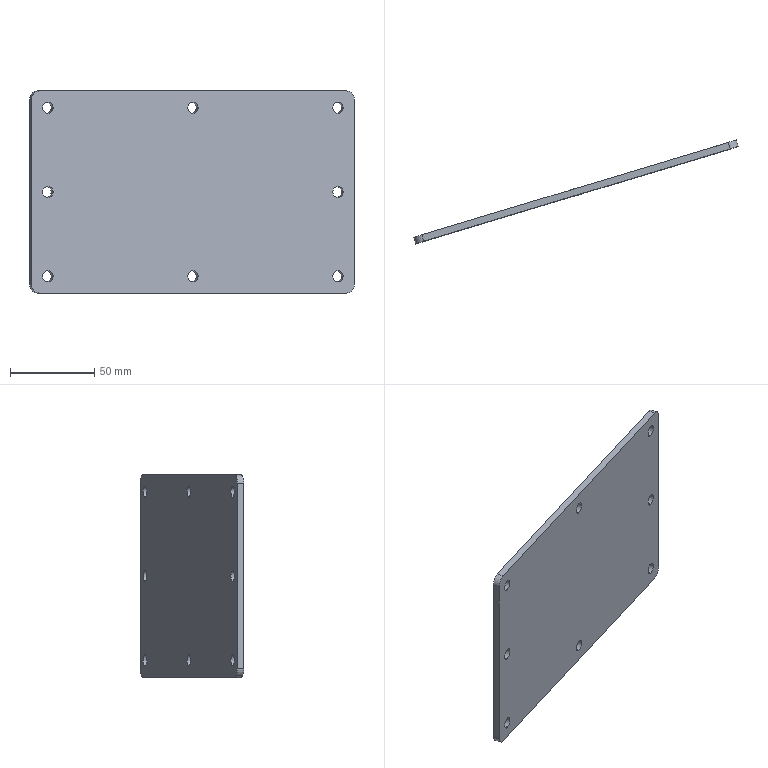Component | SolidWorks | SightHoleCoverA-1 | 1 solid | 26 faces | box 192.63 x 61.61 x 120 mm | volume 94852 mm3 | cylinder 20 | plane 6 | commonest cylinder face diameters 6.5 x16 10 x4
build123d program:
from build123d import *

# Parameters (mm, degrees)
SKETCH1_W                  = 200
SKETCH1_H                  = 120
BOSS_EXTRUDE1_DEPTH        = 4
F_6_5_6_5_DIAMETER_HOLE1_D = 6.5
FILLET1_R                  = 5


with BuildPart() as part:
    # Sketch1 → Boss-Extrude1 (new body)
    with BuildSketch(Plane(origin=(0, 0, 0), x_dir=(1, 0, 0), z_dir=(0, 1, 0))):
        Rectangle(SKETCH1_W, SKETCH1_H)
    extrude(amount=-BOSS_EXTRUDE1_DEPTH)

    # 6.5 _6.5_ Diameter Hole1 (through all)
    with Locations(Plane(origin=(0, -4, 0), x_dir=(-1, 0, 0), z_dir=(0, -1, 0))):
        with Locations((-90, 50), (0, 50), (90, 50), (90, 0), (-90, 0), (-90, -50), (0, -50), (90, -50)):
            Hole(F_6_5_6_5_DIAMETER_HOLE1_D / 2)

    # Fillet1
    fillet1_edges = [part.edges().sort_by_distance(p)[0] for p in [
        (-100, -2, 60),
        (-100, -2, -60),
        (100, -2, -60),
        (100, -2, 60),
    ]]
    fillet(fillet1_edges, radius=FILLET1_R)


solid = part.part

# Placed as in the assembly
solid = solid.moved(Location((-162.617, 165.059, 0), (180, 0, -16.791)))
STEP:
#1=COLOUR_RGB('',0.7922,0.8196,0.9333);
#2=FILL_AREA_STYLE_COLOUR('',#1);
#3=FILL_AREA_STYLE('',(#2));
#4=SURFACE_STYLE_FILL_AREA(#3);
#5=SURFACE_SIDE_STYLE('',(#4));
#6=SURFACE_STYLE_USAGE(.BOTH.,#5);
#7=PRESENTATION_STYLE_ASSIGNMENT((#6));
#8=CARTESIAN_POINT('',(-3.056,7.673,-1.841));
#9=VERTEX_POINT('',#8);
#10=CARTESIAN_POINT('',(-3.056,7.673,-2.096));
#11=VERTEX_POINT('',#10);
#12=CARTESIAN_POINT('',(-3.056,7.673,-1.969));
#13=DIRECTION('',(0.2889,-0.9574,0.));
#14=DIRECTION('',(0.,0.,-1.));
#15=AXIS2_PLACEMENT_3D('',#12,#13,#14);
#16=CIRCLE('',#15,0.128);
#17=EDGE_CURVE('',#9,#11,#16,.T.);
#18=ORIENTED_EDGE('',*,*,#17,.F.);
#19=CARTESIAN_POINT('',(-3.01,7.522,-1.841));
#20=VERTEX_POINT('',#19);
#21=CARTESIAN_POINT('',(-3.01,7.522,-1.841));
#22=DIRECTION('',(0.2889,-0.9574,0.));
#23=VECTOR('',#22,39.37);
#24=LINE('',#21,#23);
#25=EDGE_CURVE('',#9,#20,#24,.T.);
#26=ORIENTED_EDGE('',*,*,#25,.T.);
#27=CARTESIAN_POINT('',(-3.01,7.522,-2.096));
#28=VERTEX_POINT('',#27);
#29=CARTESIAN_POINT('',(-3.01,7.522,-1.969));
#30=DIRECTION('',(0.2889,-0.9574,0.));
#31=DIRECTION('',(0.,0.,-1.));
#32=AXIS2_PLACEMENT_3D('',#29,#30,#31);
#33=CIRCLE('',#32,0.128);
#34=EDGE_CURVE('',#20,#28,#33,.T.);
#35=ORIENTED_EDGE('',*,*,#34,.T.);
#36=CARTESIAN_POINT('',(-3.01,7.522,-2.096));
#37=DIRECTION('',(0.2889,-0.9574,0.));
#38=VECTOR('',#37,39.37);
#39=LINE('',#36,#38);
#40=EDGE_CURVE('',#11,#28,#39,.T.);
#41=ORIENTED_EDGE('',*,*,#40,.F.);
#42=EDGE_LOOP('',(#18,#26,#35,#41));
#43=FACE_OUTER_BOUND('',#42,.T.);
#44=CARTESIAN_POINT('',(-3.01,7.522,-1.969));
#45=DIRECTION('',(0.2889,-0.9574,0.));
#46=DIRECTION('',(0.,0.,-1.));
#47=AXIS2_PLACEMENT_3D('',#44,#45,#46);
#48=CYLINDRICAL_SURFACE('',#47,0.128);
#49=ADVANCED_FACE('',(#43),#48,.F.);
#50=CARTESIAN_POINT('',(-6.448,6.649,-1.841));
#51=VERTEX_POINT('',#50);
#52=CARTESIAN_POINT('',(-6.448,6.649,-2.096));
#53=VERTEX_POINT('',#52);
#54=CARTESIAN_POINT('',(-6.448,6.649,-1.969));
#55=DIRECTION('',(0.2889,-0.9574,0.));
#56=DIRECTION('',(0.,0.,-1.));
#57=AXIS2_PLACEMENT_3D('',#54,#55,#56);
#58=CIRCLE('',#57,0.128);
#59=EDGE_CURVE('',#51,#53,#58,.T.);
#60=ORIENTED_EDGE('',*,*,#59,.F.);
#61=CARTESIAN_POINT('',(-6.402,6.498,-1.841));
#62=VERTEX_POINT('',#61);
#63=CARTESIAN_POINT('',(-6.402,6.498,-1.841));
#64=DIRECTION('',(0.2889,-0.9574,0.));
#65=VECTOR('',#64,39.37);
#66=LINE('',#63,#65);
#67=EDGE_CURVE('',#51,#62,#66,.T.);
#68=ORIENTED_EDGE('',*,*,#67,.T.);
#69=CARTESIAN_POINT('',(-6.402,6.498,-2.096));
#70=VERTEX_POINT('',#69);
#71=CARTESIAN_POINT('',(-6.402,6.498,-1.969));
#72=DIRECTION('',(0.2889,-0.9574,0.));
#73=DIRECTION('',(0.,0.,-1.));
#74=AXIS2_PLACEMENT_3D('',#71,#72,#73);
#75=CIRCLE('',#74,0.128);
#76=EDGE_CURVE('',#62,#70,#75,.T.);
#77=ORIENTED_EDGE('',*,*,#76,.T.);
#78=CARTESIAN_POINT('',(-6.402,6.498,-2.096));
#79=DIRECTION('',(0.2889,-0.9574,0.));
#80=VECTOR('',#79,39.37);
#81=LINE('',#78,#80);
#82=EDGE_CURVE('',#53,#70,#81,.T.);
#83=ORIENTED_EDGE('',*,*,#82,.F.);
#84=EDGE_LOOP('',(#60,#68,#77,#83));
#85=FACE_OUTER_BOUND('',#84,.T.);
#86=CARTESIAN_POINT('',(-6.402,6.498,-1.969));
#87=DIRECTION('',(0.2889,-0.9574,0.));
#88=DIRECTION('',(0.,0.,-1.));
#89=AXIS2_PLACEMENT_3D('',#86,#87,#88);
#90=CYLINDRICAL_SURFACE('',#89,0.128);
#91=ADVANCED_FACE('',(#85),#90,.F.);
#92=CARTESIAN_POINT('',(-9.84,5.626,-1.841));
#93=VERTEX_POINT('',#92);
#94=CARTESIAN_POINT('',(-9.84,5.626,-2.096));
#95=VERTEX_POINT('',#94);
#96=CARTESIAN_POINT('',(-9.84,5.626,-1.969));
#97=DIRECTION('',(0.2889,-0.9574,0.));
#98=DIRECTION('',(0.,0.,-1.));
#99=AXIS2_PLACEMENT_3D('',#96,#97,#98);
#100=CIRCLE('',#99,0.128);
#101=EDGE_CURVE('',#93,#95,#100,.T.);
#102=ORIENTED_EDGE('',*,*,#101,.F.);
#103=CARTESIAN_POINT('',(-9.794,5.475,-1.841));
#104=VERTEX_POINT('',#103);
#105=CARTESIAN_POINT('',(-9.794,5.475,-1.841));
#106=DIRECTION('',(0.2889,-0.9574,0.));
#107=VECTOR('',#106,39.37);
#108=LINE('',#105,#107);
#109=EDGE_CURVE('',#93,#104,#108,.T.);
#110=ORIENTED_EDGE('',*,*,#109,.T.);
#111=CARTESIAN_POINT('',(-9.794,5.475,-2.096));
#112=VERTEX_POINT('',#111);
#113=CARTESIAN_POINT('',(-9.794,5.475,-1.969));
#114=DIRECTION('',(0.2889,-0.9574,0.));
#115=DIRECTION('',(0.,0.,-1.));
#116=AXIS2_PLACEMENT_3D('',#113,#114,#115);
#117=CIRCLE('',#116,0.128);
#118=EDGE_CURVE('',#104,#112,#117,.T.);
#119=ORIENTED_EDGE('',*,*,#118,.T.);
#120=CARTESIAN_POINT('',(-9.794,5.475,-2.096));
#121=DIRECTION('',(0.2889,-0.9574,0.));
#122=VECTOR('',#121,39.37);
#123=LINE('',#120,#122);
#124=EDGE_CURVE('',#95,#112,#123,.T.);
#125=ORIENTED_EDGE('',*,*,#124,.F.);
#126=EDGE_LOOP('',(#102,#110,#119,#125));
#127=FACE_OUTER_BOUND('',#126,.T.);
#128=CARTESIAN_POINT('',(-9.794,5.475,-1.969));
#129=DIRECTION('',(0.2889,-0.9574,0.));
#130=DIRECTION('',(0.,0.,-1.));
#131=AXIS2_PLACEMENT_3D('',#128,#129,#130);
#132=CYLINDRICAL_SURFACE('',#131,0.128);
#133=ADVANCED_FACE('',(#127),#132,.F.);
#134=CARTESIAN_POINT('',(-9.84,5.626,0.128));
#135=VERTEX_POINT('',#134);
#136=CARTESIAN_POINT('',(-9.84,5.626,-0.128));
#137=VERTEX_POINT('',#136);
#138=CARTESIAN_POINT('',(-9.84,5.626,0.));
#139=DIRECTION('',(0.2889,-0.9574,0.));
#140=DIRECTION('',(0.,0.,-1.));
#141=AXIS2_PLACEMENT_3D('',#138,#139,#140);
#142=CIRCLE('',#141,0.128);
#143=EDGE_CURVE('',#135,#137,#142,.T.);
#144=ORIENTED_EDGE('',*,*,#143,.F.);
#145=CARTESIAN_POINT('',(-9.794,5.475,0.128));
#146=VERTEX_POINT('',#145);
#147=CARTESIAN_POINT('',(-9.794,5.475,0.128));
#148=DIRECTION('',(0.2889,-0.9574,0.));
#149=VECTOR('',#148,39.37);
#150=LINE('',#147,#149);
#151=EDGE_CURVE('',#135,#146,#150,.T.);
#152=ORIENTED_EDGE('',*,*,#151,.T.);
#153=CARTESIAN_POINT('',(-9.794,5.475,-0.128));
#154=VERTEX_POINT('',#153);
#155=CARTESIAN_POINT('',(-9.794,5.475,0.));
#156=DIRECTION('',(0.2889,-0.9574,0.));
#157=DIRECTION('',(0.,0.,-1.));
#158=AXIS2_PLACEMENT_3D('',#155,#156,#157);
#159=CIRCLE('',#158,0.128);
#160=EDGE_CURVE('',#146,#154,#159,.T.);
#161=ORIENTED_EDGE('',*,*,#160,.T.);
#162=CARTESIAN_POINT('',(-9.794,5.475,-0.128));
#163=DIRECTION('',(0.2889,-0.9574,0.));
#164=VECTOR('',#163,39.37);
#165=LINE('',#162,#164);
#166=EDGE_CURVE('',#137,#154,#165,.T.);
#167=ORIENTED_EDGE('',*,*,#166,.F.);
#168=EDGE_LOOP('',(#144,#152,#161,#167));
#169=FACE_OUTER_BOUND('',#168,.T.);
#170=CARTESIAN_POINT('',(-9.794,5.475,0.));
#171=DIRECTION('',(0.2889,-0.9574,0.));
#172=DIRECTION('',(0.,0.,-1.));
#173=AXIS2_PLACEMENT_3D('',#170,#171,#172);
#174=CYLINDRICAL_SURFACE('',#173,0.128);
#175=ADVANCED_FACE('',(#169),#174,.F.);
#176=CARTESIAN_POINT('',(-3.056,7.673,0.128));
#177=VERTEX_POINT('',#176);
#178=CARTESIAN_POINT('',(-3.056,7.673,-0.128));
#179=VERTEX_POINT('',#178);
#180=CARTESIAN_POINT('',(-3.056,7.673,0.));
#181=DIRECTION('',(0.2889,-0.9574,0.));
#182=DIRECTION('',(0.,0.,-1.));
#183=AXIS2_PLACEMENT_3D('',#180,#181,#182);
#184=CIRCLE('',#183,0.128);
#185=EDGE_CURVE('',#177,#179,#184,.T.);
#186=ORIENTED_EDGE('',*,*,#185,.F.);
#187=CARTESIAN_POINT('',(-3.01,7.522,0.128));
#188=VERTEX_POINT('',#187);
#189=CARTESIAN_POINT('',(-3.01,7.522,0.128));
#190=DIRECTION('',(0.2889,-0.9574,0.));
#191=VECTOR('',#190,39.37);
#192=LINE('',#189,#191);
#193=EDGE_CURVE('',#177,#188,#192,.T.);
#194=ORIENTED_EDGE('',*,*,#193,.T.);
#195=CARTESIAN_POINT('',(-3.01,7.522,-0.128));
#196=VERTEX_POINT('',#195);
#197=CARTESIAN_POINT('',(-3.01,7.522,0.));
#198=DIRECTION('',(0.2889,-0.9574,0.));
#199=DIRECTION('',(0.,0.,-1.));
#200=AXIS2_PLACEMENT_3D('',#197,#198,#199);
#201=CIRCLE('',#200,0.128);
#202=EDGE_CURVE('',#188,#196,#201,.T.);
#203=ORIENTED_EDGE('',*,*,#202,.T.);
#204=CARTESIAN_POINT('',(-3.01,7.522,-0.128));
#205=DIRECTION('',(0.2889,-0.9574,0.));
#206=VECTOR('',#205,39.37);
#207=LINE('',#204,#206);
#208=EDGE_CURVE('',#179,#196,#207,.T.);
#209=ORIENTED_EDGE('',*,*,#208,.F.);
#210=EDGE_LOOP('',(#186,#194,#203,#209));
#211=FACE_OUTER_BOUND('',#210,.T.);
#212=CARTESIAN_POINT('',(-3.01,7.522,0.));
#213=DIRECTION('',(0.2889,-0.9574,0.));
#214=DIRECTION('',(0.,0.,-1.));
#215=AXIS2_PLACEMENT_3D('',#212,#213,#214);
#216=CYLINDRICAL_SURFACE('',#215,0.128);
#217=ADVANCED_FACE('',(#211),#216,.F.);
#218=CARTESIAN_POINT('',(-3.056,7.673,2.096));
#219=VERTEX_POINT('',#218);
#220=CARTESIAN_POINT('',(-3.056,7.673,1.841));
#221=VERTEX_POINT('',#220);
#222=CARTESIAN_POINT('',(-3.056,7.673,1.969));
#223=DIRECTION('',(0.2889,-0.9574,0.));
#224=DIRECTION('',(0.,0.,-1.));
#225=AXIS2_PLACEMENT_3D('',#222,#223,#224);
#226=CIRCLE('',#225,0.128);
#227=EDGE_CURVE('',#219,#221,#226,.T.);
#228=ORIENTED_EDGE('',*,*,#227,.F.);
#229=CARTESIAN_POINT('',(-3.01,7.522,2.096));
#230=VERTEX_POINT('',#229);
#231=CARTESIAN_POINT('',(-3.01,7.522,2.096));
#232=DIRECTION('',(0.2889,-0.9574,0.));
#233=VECTOR('',#232,39.37);
#234=LINE('',#231,#233);
#235=EDGE_CURVE('',#219,#230,#234,.T.);
#236=ORIENTED_EDGE('',*,*,#235,.T.);
#237=CARTESIAN_POINT('',(-3.01,7.522,1.841));
#238=VERTEX_POINT('',#237);
#239=CARTESIAN_POINT('',(-3.01,7.522,1.969));
#240=DIRECTION('',(0.2889,-0.9574,0.));
#241=DIRECTION('',(0.,0.,-1.));
#242=AXIS2_PLACEMENT_3D('',#239,#240,#241);
#243=CIRCLE('',#242,0.128);
#244=EDGE_CURVE('',#230,#238,#243,.T.);
#245=ORIENTED_EDGE('',*,*,#244,.T.);
#246=CARTESIAN_POINT('',(-3.01,7.522,1.841));
#247=DIRECTION('',(0.2889,-0.9574,0.));
#248=VECTOR('',#247,39.37);
#249=LINE('',#246,#248);
#250=EDGE_CURVE('',#221,#238,#249,.T.);
#251=ORIENTED_EDGE('',*,*,#250,.F.);
#252=EDGE_LOOP('',(#228,#236,#245,#251));
#253=FACE_OUTER_BOUND('',#252,.T.);
#254=CARTESIAN_POINT('',(-3.01,7.522,1.969));
#255=DIRECTION('',(0.2889,-0.9574,0.));
#256=DIRECTION('',(0.,0.,-1.));
#257=AXIS2_PLACEMENT_3D('',#254,#255,#256);
#258=CYLINDRICAL_SURFACE('',#257,0.128);
#259=ADVANCED_FACE('',(#253),#258,.F.);
#260=CARTESIAN_POINT('',(-6.448,6.649,2.096));
#261=VERTEX_POINT('',#260);
#262=CARTESIAN_POINT('',(-6.448,6.649,1.841));
#263=VERTEX_POINT('',#262);
#264=CARTESIAN_POINT('',(-6.448,6.649,1.969));
#265=DIRECTION('',(0.2889,-0.9574,0.));
#266=DIRECTION('',(0.,0.,-1.));
#267=AXIS2_PLACEMENT_3D('',#264,#265,#266);
#268=CIRCLE('',#267,0.128);
#269=EDGE_CURVE('',#261,#263,#268,.T.);
#270=ORIENTED_EDGE('',*,*,#269,.F.);
#271=CARTESIAN_POINT('',(-6.402,6.498,2.096));
#272=VERTEX_POINT('',#271);
#273=CARTESIAN_POINT('',(-6.402,6.498,2.096));
#274=DIRECTION('',(0.2889,-0.9574,0.));
#275=VECTOR('',#274,39.37);
#276=LINE('',#273,#275);
#277=EDGE_CURVE('',#261,#272,#276,.T.);
#278=ORIENTED_EDGE('',*,*,#277,.T.);
#279=CARTESIAN_POINT('',(-6.402,6.498,1.841));
#280=VERTEX_POINT('',#279);
#281=CARTESIAN_POINT('',(-6.402,6.498,1.969));
#282=DIRECTION('',(0.2889,-0.9574,0.));
#283=DIRECTION('',(0.,0.,-1.));
#284=AXIS2_PLACEMENT_3D('',#281,#282,#283);
#285=CIRCLE('',#284,0.128);
#286=EDGE_CURVE('',#272,#280,#285,.T.);
#287=ORIENTED_EDGE('',*,*,#286,.T.);
#288=CARTESIAN_POINT('',(-6.402,6.498,1.841));
#289=DIRECTION('',(0.2889,-0.9574,0.));
#290=VECTOR('',#289,39.37);
#291=LINE('',#288,#290);
#292=EDGE_CURVE('',#263,#280,#291,.T.);
#293=ORIENTED_EDGE('',*,*,#292,.F.);
#294=EDGE_LOOP('',(#270,#278,#287,#293));
#295=FACE_OUTER_BOUND('',#294,.T.);
#296=CARTESIAN_POINT('',(-6.402,6.498,1.969));
#297=DIRECTION('',(0.2889,-0.9574,0.));
#298=DIRECTION('',(0.,0.,-1.));
#299=AXIS2_PLACEMENT_3D('',#296,#297,#298);
#300=CYLINDRICAL_SURFACE('',#299,0.128);
#301=ADVANCED_FACE('',(#295),#300,.F.);
#302=CARTESIAN_POINT('',(-9.84,5.626,2.096));
#303=VERTEX_POINT('',#302);
#304=CARTESIAN_POINT('',(-9.84,5.626,1.841));
#305=VERTEX_POINT('',#304);
#306=CARTESIAN_POINT('',(-9.84,5.626,1.969));
#307=DIRECTION('',(0.2889,-0.9574,0.));
#308=DIRECTION('',(0.,0.,-1.));
#309=AXIS2_PLACEMENT_3D('',#306,#307,#308);
#310=CIRCLE('',#309,0.128);
#311=EDGE_CURVE('',#303,#305,#310,.T.);
#312=ORIENTED_EDGE('',*,*,#311,.F.);
#313=CARTESIAN_POINT('',(-9.794,5.475,2.096));
#314=VERTEX_POINT('',#313);
#315=CARTESIAN_POINT('',(-9.794,5.475,2.096));
#316=DIRECTION('',(0.2889,-0.9574,0.));
#317=VECTOR('',#316,39.37);
#318=LINE('',#315,#317);
#319=EDGE_CURVE('',#303,#314,#318,.T.);
#320=ORIENTED_EDGE('',*,*,#319,.T.);
#321=CARTESIAN_POINT('',(-9.794,5.475,1.841));
#322=VERTEX_POINT('',#321);
#323=CARTESIAN_POINT('',(-9.794,5.475,1.969));
#324=DIRECTION('',(0.2889,-0.9574,0.));
#325=DIRECTION('',(0.,0.,-1.));
#326=AXIS2_PLACEMENT_3D('',#323,#324,#325);
#327=CIRCLE('',#326,0.128);
#328=EDGE_CURVE('',#314,#322,#327,.T.);
#329=ORIENTED_EDGE('',*,*,#328,.T.);
#330=CARTESIAN_POINT('',(-9.794,5.475,1.841));
#331=DIRECTION('',(0.2889,-0.9574,0.));
#332=VECTOR('',#331,39.37);
#333=LINE('',#330,#332);
#334=EDGE_CURVE('',#305,#322,#333,.T.);
#335=ORIENTED_EDGE('',*,*,#334,.F.);
#336=EDGE_LOOP('',(#312,#320,#329,#335));
#337=FACE_OUTER_BOUND('',#336,.T.);
#338=CARTESIAN_POINT('',(-9.794,5.475,1.969));
#339=DIRECTION('',(0.2889,-0.9574,0.));
#340=DIRECTION('',(0.,0.,-1.));
#341=AXIS2_PLACEMENT_3D('',#338,#339,#340);
#342=CYLINDRICAL_SURFACE('',#341,0.128);
#343=ADVANCED_FACE('',(#337),#342,.F.);
#344=CARTESIAN_POINT('',(-3.056,7.673,-1.969));
#345=DIRECTION('',(0.2889,-0.9574,0.));
#346=DIRECTION('',(0.,0.,-1.));
#347=AXIS2_PLACEMENT_3D('',#344,#345,#346);
#348=CIRCLE('',#347,0.128);
#349=EDGE_CURVE('',#11,#9,#348,.T.);
#350=ORIENTED_EDGE('',*,*,#349,.T.);
#351=ORIENTED_EDGE('',*,*,#17,.T.);
#352=EDGE_LOOP('',(#350,#351));
#353=FACE_BOUND('',#352,.T.);
#354=CARTESIAN_POINT('',(-10.028,5.569,2.362));
#355=VERTEX_POINT('',#354);
#356=CARTESIAN_POINT('',(-2.867,7.73,2.362));
#357=VERTEX_POINT('',#356);
#358=CARTESIAN_POINT('',(-10.217,5.512,2.362));
#359=DIRECTION('',(0.9574,0.2889,0.));
#360=VECTOR('',#359,39.37);
#361=LINE('',#358,#360);
#362=EDGE_CURVE('',#355,#357,#361,.T.);
#363=ORIENTED_EDGE('',*,*,#362,.T.);
#364=CARTESIAN_POINT('',(-2.679,7.787,2.165));
#365=VERTEX_POINT('',#364);
#366=CARTESIAN_POINT('',(-2.867,7.73,2.165));
#367=DIRECTION('',(-0.2889,0.9574,0.));
#368=DIRECTION('',(0.,0.,1.));
#369=AXIS2_PLACEMENT_3D('',#366,#367,#368);
#370=CIRCLE('',#369,0.1969);
#371=EDGE_CURVE('',#357,#365,#370,.T.);
#372=ORIENTED_EDGE('',*,*,#371,.T.);
#373=CARTESIAN_POINT('',(-2.679,7.787,-2.165));
#374=VERTEX_POINT('',#373);
#375=CARTESIAN_POINT('',(-2.679,7.787,2.362));
#376=DIRECTION('',(0.,0.,-1.));
#377=VECTOR('',#376,39.37);
#378=LINE('',#375,#377);
#379=EDGE_CURVE('',#365,#374,#378,.T.);
#380=ORIENTED_EDGE('',*,*,#379,.T.);
#381=CARTESIAN_POINT('',(-2.867,7.73,-2.362));
#382=VERTEX_POINT('',#381);
#383=CARTESIAN_POINT('',(-2.867,7.73,-2.165));
#384=DIRECTION('',(-0.2889,0.9574,0.));
#385=DIRECTION('',(0.,0.,1.));
#386=AXIS2_PLACEMENT_3D('',#383,#384,#385);
#387=CIRCLE('',#386,0.1969);
#388=EDGE_CURVE('',#374,#382,#387,.T.);
#389=ORIENTED_EDGE('',*,*,#388,.T.);
#390=CARTESIAN_POINT('',(-10.028,5.569,-2.362));
#391=VERTEX_POINT('',#390);
#392=CARTESIAN_POINT('',(-2.679,7.787,-2.362));
#393=DIRECTION('',(-0.9574,-0.2889,0.));
#394=VECTOR('',#393,39.37);
#395=LINE('',#392,#394);
#396=EDGE_CURVE('',#382,#391,#395,.T.);
#397=ORIENTED_EDGE('',*,*,#396,.T.);
#398=CARTESIAN_POINT('',(-10.217,5.512,-2.165));
#399=VERTEX_POINT('',#398);
#400=CARTESIAN_POINT('',(-10.028,5.569,-2.165));
#401=DIRECTION('',(-0.2889,0.9574,0.));
#402=DIRECTION('',(0.,0.,1.));
#403=AXIS2_PLACEMENT_3D('',#400,#401,#402);
#404=CIRCLE('',#403,0.1969);
#405=EDGE_CURVE('',#391,#399,#404,.T.);
#406=ORIENTED_EDGE('',*,*,#405,.T.);
#407=CARTESIAN_POINT('',(-10.217,5.512,2.165));
#408=VERTEX_POINT('',#407);
#409=CARTESIAN_POINT('',(-10.217,5.512,-2.362));
#410=DIRECTION('',(-0.,-0.,1.));
#411=VECTOR('',#410,39.37);
#412=LINE('',#409,#411);
#413=EDGE_CURVE('',#399,#408,#412,.T.);
#414=ORIENTED_EDGE('',*,*,#413,.T.);
#415=CARTESIAN_POINT('',(-10.028,5.569,2.165));
#416=DIRECTION('',(-0.2889,0.9574,0.));
#417=DIRECTION('',(0.,0.,1.));
#418=AXIS2_PLACEMENT_3D('',#415,#416,#417);
#419=CIRCLE('',#418,0.1969);
#420=EDGE_CURVE('',#408,#355,#419,.T.);
#421=ORIENTED_EDGE('',*,*,#420,.T.);
#422=EDGE_LOOP('',(#363,#372,#380,#389,#397,#406,#414,#421));
#423=FACE_OUTER_BOUND('',#422,.T.);
#424=CARTESIAN_POINT('',(-9.84,5.626,1.969));
#425=DIRECTION('',(0.2889,-0.9574,0.));
#426=DIRECTION('',(0.,0.,-1.));
#427=AXIS2_PLACEMENT_3D('',#424,#425,#426);
#428=CIRCLE('',#427,0.128);
#429=EDGE_CURVE('',#305,#303,#428,.T.);
#430=ORIENTED_EDGE('',*,*,#429,.T.);
#431=ORIENTED_EDGE('',*,*,#311,.T.);
#432=EDGE_LOOP('',(#430,#431));
#433=FACE_BOUND('',#432,.T.);
#434=CARTESIAN_POINT('',(-6.448,6.649,1.969));
#435=DIRECTION('',(0.2889,-0.9574,0.));
#436=DIRECTION('',(0.,0.,-1.));
#437=AXIS2_PLACEMENT_3D('',#434,#435,#436);
#438=CIRCLE('',#437,0.128);
#439=EDGE_CURVE('',#263,#261,#438,.T.);
#440=ORIENTED_EDGE('',*,*,#439,.T.);
#441=ORIENTED_EDGE('',*,*,#269,.T.);
#442=EDGE_LOOP('',(#440,#441));
#443=FACE_BOUND('',#442,.T.);
#444=CARTESIAN_POINT('',(-3.056,7.673,1.969));
#445=DIRECTION('',(0.2889,-0.9574,0.));
#446=DIRECTION('',(0.,0.,-1.));
#447=AXIS2_PLACEMENT_3D('',#444,#445,#446);
#448=CIRCLE('',#447,0.128);
#449=EDGE_CURVE('',#221,#219,#448,.T.);
#450=ORIENTED_EDGE('',*,*,#449,.T.);
#451=ORIENTED_EDGE('',*,*,#227,.T.);
#452=EDGE_LOOP('',(#450,#451));
#453=FACE_BOUND('',#452,.T.);
#454=CARTESIAN_POINT('',(-3.056,7.673,0.));
#455=DIRECTION('',(0.2889,-0.9574,0.));
#456=DIRECTION('',(0.,0.,-1.));
#457=AXIS2_PLACEMENT_3D('',#454,#455,#456);
#458=CIRCLE('',#457,0.128);
#459=EDGE_CURVE('',#179,#177,#458,.T.);
#460=ORIENTED_EDGE('',*,*,#459,.T.);
#461=ORIENTED_EDGE('',*,*,#185,.T.);
#462=EDGE_LOOP('',(#460,#461));
#463=FACE_BOUND('',#462,.T.);
#464=CARTESIAN_POINT('',(-9.84,5.626,0.));
#465=DIRECTION('',(0.2889,-0.9574,0.));
#466=DIRECTION('',(0.,0.,-1.));
#467=AXIS2_PLACEMENT_3D('',#464,#465,#466);
#468=CIRCLE('',#467,0.128);
#469=EDGE_CURVE('',#137,#135,#468,.T.);
#470=ORIENTED_EDGE('',*,*,#469,.T.);
#471=ORIENTED_EDGE('',*,*,#143,.T.);
#472=EDGE_LOOP('',(#470,#471));
#473=FACE_BOUND('',#472,.T.);
#474=CARTESIAN_POINT('',(-9.84,5.626,-1.969));
#475=DIRECTION('',(0.2889,-0.9574,0.));
#476=DIRECTION('',(0.,0.,-1.));
#477=AXIS2_PLACEMENT_3D('',#474,#475,#476);
#478=CIRCLE('',#477,0.128);
#479=EDGE_CURVE('',#95,#93,#478,.T.);
#480=ORIENTED_EDGE('',*,*,#479,.T.);
#481=ORIENTED_EDGE('',*,*,#101,.T.);
#482=EDGE_LOOP('',(#480,#481));
#483=FACE_BOUND('',#482,.T.);
#484=CARTESIAN_POINT('',(-6.448,6.649,-1.969));
#485=DIRECTION('',(0.2889,-0.9574,0.));
#486=DIRECTION('',(0.,0.,-1.));
#487=AXIS2_PLACEMENT_3D('',#484,#485,#486);
#488=CIRCLE('',#487,0.128);
#489=EDGE_CURVE('',#53,#51,#488,.T.);
#490=ORIENTED_EDGE('',*,*,#489,.T.);
#491=ORIENTED_EDGE('',*,*,#59,.T.);
#492=EDGE_LOOP('',(#490,#491));
#493=FACE_BOUND('',#492,.T.);
#494=CARTESIAN_POINT('',(-6.448,6.649,0.));
#495=DIRECTION('',(-0.2889,0.9574,0.));
#496=DIRECTION('',(0.,0.,1.));
#497=AXIS2_PLACEMENT_3D('',#494,#495,#496);
#498=PLANE('',#497);
#499=ADVANCED_FACE('',(#353,#423,#433,#443,#453,#463,#473,#483,#493),#498,.T.);
#500=CARTESIAN_POINT('',(-9.983,5.418,2.362));
#501=VERTEX_POINT('',#500);
#502=CARTESIAN_POINT('',(-2.822,7.579,2.362));
#503=VERTEX_POINT('',#502);
#504=CARTESIAN_POINT('',(-10.171,5.361,2.362));
#505=DIRECTION('',(0.9574,0.2889,0.));
#506=VECTOR('',#505,39.37);
#507=LINE('',#504,#506);
#508=EDGE_CURVE('',#501,#503,#507,.T.);
#509=ORIENTED_EDGE('',*,*,#508,.T.);
#510=CARTESIAN_POINT('',(-2.822,7.579,2.362));
#511=DIRECTION('',(-0.2889,0.9574,0.));
#512=VECTOR('',#511,39.37);
#513=LINE('',#510,#512);
#514=EDGE_CURVE('',#503,#357,#513,.T.);
#515=ORIENTED_EDGE('',*,*,#514,.T.);
#516=ORIENTED_EDGE('',*,*,#362,.F.);
#517=CARTESIAN_POINT('',(-9.983,5.418,2.362));
#518=DIRECTION('',(0.2889,-0.9574,0.));
#519=VECTOR('',#518,39.37);
#520=LINE('',#517,#519);
#521=EDGE_CURVE('',#355,#501,#520,.T.);
#522=ORIENTED_EDGE('',*,*,#521,.T.);
#523=EDGE_LOOP('',(#509,#515,#516,#522));
#524=FACE_OUTER_BOUND('',#523,.T.);
#525=CARTESIAN_POINT('',(-10.171,5.361,2.362));
#526=DIRECTION('',(0.,0.,1.));
#527=DIRECTION('',(0.9574,0.2889,0.));
#528=AXIS2_PLACEMENT_3D('',#525,#526,#527);
#529=PLANE('',#528);
#530=ADVANCED_FACE('',(#524),#529,.T.);
#531=CARTESIAN_POINT('',(-10.171,5.361,-2.165));
#532=VERTEX_POINT('',#531);
#533=CARTESIAN_POINT('',(-10.171,5.361,2.165));
#534=VERTEX_POINT('',#533);
#535=CARTESIAN_POINT('',(-10.171,5.361,-2.362));
#536=DIRECTION('',(-0.,-0.,1.));
#537=VECTOR('',#536,39.37);
#538=LINE('',#535,#537);
#539=EDGE_CURVE('',#532,#534,#538,.T.);
#540=ORIENTED_EDGE('',*,*,#539,.T.);
#541=CARTESIAN_POINT('',(-10.171,5.361,2.165));
#542=DIRECTION('',(-0.2889,0.9574,0.));
#543=VECTOR('',#542,39.37);
#544=LINE('',#541,#543);
#545=EDGE_CURVE('',#534,#408,#544,.T.);
#546=ORIENTED_EDGE('',*,*,#545,.T.);
#547=ORIENTED_EDGE('',*,*,#413,.F.);
#548=CARTESIAN_POINT('',(-10.171,5.361,-2.165));
#549=DIRECTION('',(0.2889,-0.9574,0.));
#550=VECTOR('',#549,39.37);
#551=LINE('',#548,#550);
#552=EDGE_CURVE('',#399,#532,#551,.T.);
#553=ORIENTED_EDGE('',*,*,#552,.T.);
#554=EDGE_LOOP('',(#540,#546,#547,#553));
#555=FACE_OUTER_BOUND('',#554,.T.);
#556=CARTESIAN_POINT('',(-10.171,5.361,-2.362));
#557=DIRECTION('',(-0.9574,-0.2889,-0.));
#558=DIRECTION('',(-0.,-0.,1.));
#559=AXIS2_PLACEMENT_3D('',#556,#557,#558);
#560=PLANE('',#559);
#561=ADVANCED_FACE('',(#555),#560,.T.);
#562=ORIENTED_EDGE('',*,*,#396,.F.);
#563=CARTESIAN_POINT('',(-2.822,7.579,-2.362));
#564=VERTEX_POINT('',#563);
#565=CARTESIAN_POINT('',(-2.822,7.579,-2.362));
#566=DIRECTION('',(0.2889,-0.9574,0.));
#567=VECTOR('',#566,39.37);
#568=LINE('',#565,#567);
#569=EDGE_CURVE('',#382,#564,#568,.T.);
#570=ORIENTED_EDGE('',*,*,#569,.T.);
#571=CARTESIAN_POINT('',(-9.983,5.418,-2.362));
#572=VERTEX_POINT('',#571);
#573=CARTESIAN_POINT('',(-2.633,7.636,-2.362));
#574=DIRECTION('',(-0.9574,-0.2889,0.));
#575=VECTOR('',#574,39.37);
#576=LINE('',#573,#575);
#577=EDGE_CURVE('',#564,#572,#576,.T.);
#578=ORIENTED_EDGE('',*,*,#577,.T.);
#579=CARTESIAN_POINT('',(-9.983,5.418,-2.362));
#580=DIRECTION('',(-0.2889,0.9574,0.));
#581=VECTOR('',#580,39.37);
#582=LINE('',#579,#581);
#583=EDGE_CURVE('',#572,#391,#582,.T.);
#584=ORIENTED_EDGE('',*,*,#583,.T.);
#585=EDGE_LOOP('',(#562,#570,#578,#584));
#586=FACE_OUTER_BOUND('',#585,.T.);
#587=CARTESIAN_POINT('',(-2.633,7.636,-2.362));
#588=DIRECTION('',(-0.,-0.,-1.));
#589=DIRECTION('',(-0.9574,-0.2889,0.));
#590=AXIS2_PLACEMENT_3D('',#587,#588,#589);
#591=PLANE('',#590);
#592=ADVANCED_FACE('',(#586),#591,.T.);
#593=ORIENTED_EDGE('',*,*,#379,.F.);
#594=CARTESIAN_POINT('',(-2.633,7.636,2.165));
#595=VERTEX_POINT('',#594);
#596=CARTESIAN_POINT('',(-2.633,7.636,2.165));
#597=DIRECTION('',(0.2889,-0.9574,0.));
#598=VECTOR('',#597,39.37);
#599=LINE('',#596,#598);
#600=EDGE_CURVE('',#365,#595,#599,.T.);
#601=ORIENTED_EDGE('',*,*,#600,.T.);
#602=CARTESIAN_POINT('',(-2.633,7.636,-2.165));
#603=VERTEX_POINT('',#602);
#604=CARTESIAN_POINT('',(-2.633,7.636,2.362));
#605=DIRECTION('',(0.,0.,-1.));
#606=VECTOR('',#605,39.37);
#607=LINE('',#604,#606);
#608=EDGE_CURVE('',#595,#603,#607,.T.);
#609=ORIENTED_EDGE('',*,*,#608,.T.);
#610=CARTESIAN_POINT('',(-2.633,7.636,-2.165));
#611=DIRECTION('',(-0.2889,0.9574,0.));
#612=VECTOR('',#611,39.37);
#613=LINE('',#610,#612);
#614=EDGE_CURVE('',#603,#374,#613,.T.);
#615=ORIENTED_EDGE('',*,*,#614,.T.);
#616=EDGE_LOOP('',(#593,#601,#609,#615));
#617=FACE_OUTER_BOUND('',#616,.T.);
#618=CARTESIAN_POINT('',(-2.633,7.636,2.362));
#619=DIRECTION('',(0.9574,0.2889,0.));
#620=DIRECTION('',(0.,0.,-1.));
#621=AXIS2_PLACEMENT_3D('',#618,#619,#620);
#622=PLANE('',#621);
#623=ADVANCED_FACE('',(#617),#622,.T.);
#624=CARTESIAN_POINT('',(-3.01,7.522,-1.969));
#625=DIRECTION('',(0.2889,-0.9574,0.));
#626=DIRECTION('',(0.,0.,-1.));
#627=AXIS2_PLACEMENT_3D('',#624,#625,#626);
#628=CIRCLE('',#627,0.128);
#629=EDGE_CURVE('',#28,#20,#628,.T.);
#630=ORIENTED_EDGE('',*,*,#629,.F.);
#631=ORIENTED_EDGE('',*,*,#34,.F.);
#632=EDGE_LOOP('',(#630,#631));
#633=FACE_BOUND('',#632,.T.);
#634=CARTESIAN_POINT('',(-6.402,6.498,-1.969));
#635=DIRECTION('',(0.2889,-0.9574,0.));
#636=DIRECTION('',(0.,0.,-1.));
#637=AXIS2_PLACEMENT_3D('',#634,#635,#636);
#638=CIRCLE('',#637,0.128);
#639=EDGE_CURVE('',#70,#62,#638,.T.);
#640=ORIENTED_EDGE('',*,*,#639,.F.);
#641=ORIENTED_EDGE('',*,*,#76,.F.);
#642=EDGE_LOOP('',(#640,#641));
#643=FACE_BOUND('',#642,.T.);
#644=CARTESIAN_POINT('',(-9.794,5.475,-1.969));
#645=DIRECTION('',(0.2889,-0.9574,0.));
#646=DIRECTION('',(0.,0.,-1.));
#647=AXIS2_PLACEMENT_3D('',#644,#645,#646);
#648=CIRCLE('',#647,0.128);
#649=EDGE_CURVE('',#112,#104,#648,.T.);
#650=ORIENTED_EDGE('',*,*,#649,.F.);
#651=ORIENTED_EDGE('',*,*,#118,.F.);
#652=EDGE_LOOP('',(#650,#651));
#653=FACE_BOUND('',#652,.T.);
#654=CARTESIAN_POINT('',(-9.794,5.475,0.));
#655=DIRECTION('',(0.2889,-0.9574,0.));
#656=DIRECTION('',(0.,0.,-1.));
#657=AXIS2_PLACEMENT_3D('',#654,#655,#656);
#658=CIRCLE('',#657,0.128);
#659=EDGE_CURVE('',#154,#146,#658,.T.);
#660=ORIENTED_EDGE('',*,*,#659,.F.);
#661=ORIENTED_EDGE('',*,*,#160,.F.);
#662=EDGE_LOOP('',(#660,#661));
#663=FACE_BOUND('',#662,.T.);
#664=CARTESIAN_POINT('',(-3.01,7.522,0.));
#665=DIRECTION('',(0.2889,-0.9574,0.));
#666=DIRECTION('',(0.,0.,-1.));
#667=AXIS2_PLACEMENT_3D('',#664,#665,#666);
#668=CIRCLE('',#667,0.128);
#669=EDGE_CURVE('',#196,#188,#668,.T.);
#670=ORIENTED_EDGE('',*,*,#669,.F.);
#671=ORIENTED_EDGE('',*,*,#202,.F.);
#672=EDGE_LOOP('',(#670,#671));
#673=FACE_BOUND('',#672,.T.);
#674=CARTESIAN_POINT('',(-3.01,7.522,1.969));
#675=DIRECTION('',(0.2889,-0.9574,0.));
#676=DIRECTION('',(0.,0.,-1.));
#677=AXIS2_PLACEMENT_3D('',#674,#675,#676);
#678=CIRCLE('',#677,0.128);
#679=EDGE_CURVE('',#238,#230,#678,.T.);
#680=ORIENTED_EDGE('',*,*,#679,.F.);
#681=ORIENTED_EDGE('',*,*,#244,.F.);
#682=EDGE_LOOP('',(#680,#681));
#683=FACE_BOUND('',#682,.T.);
#684=CARTESIAN_POINT('',(-6.402,6.498,1.969));
#685=DIRECTION('',(0.2889,-0.9574,0.));
#686=DIRECTION('',(0.,0.,-1.));
#687=AXIS2_PLACEMENT_3D('',#684,#685,#686);
#688=CIRCLE('',#687,0.128);
#689=EDGE_CURVE('',#280,#272,#688,.T.);
#690=ORIENTED_EDGE('',*,*,#689,.F.);
#691=ORIENTED_EDGE('',*,*,#286,.F.);
#692=EDGE_LOOP('',(#690,#691));
#693=FACE_BOUND('',#692,.T.);
#694=CARTESIAN_POINT('',(-9.794,5.475,1.969));
#695=DIRECTION('',(0.2889,-0.9574,0.));
#696=DIRECTION('',(0.,0.,-1.));
#697=AXIS2_PLACEMENT_3D('',#694,#695,#696);
#698=CIRCLE('',#697,0.128);
#699=EDGE_CURVE('',#322,#314,#698,.T.);
#700=ORIENTED_EDGE('',*,*,#699,.F.);
#701=ORIENTED_EDGE('',*,*,#328,.F.);
#702=EDGE_LOOP('',(#700,#701));
#703=FACE_BOUND('',#702,.T.);
#704=ORIENTED_EDGE('',*,*,#608,.F.);
#705=CARTESIAN_POINT('',(-2.822,7.579,2.165));
#706=DIRECTION('',(0.2889,-0.9574,0.));
#707=DIRECTION('',(0.,0.,1.));
#708=AXIS2_PLACEMENT_3D('',#705,#706,#707);
#709=CIRCLE('',#708,0.1969);
#710=EDGE_CURVE('',#595,#503,#709,.T.);
#711=ORIENTED_EDGE('',*,*,#710,.T.);
#712=ORIENTED_EDGE('',*,*,#508,.F.);
#713=CARTESIAN_POINT('',(-9.983,5.418,2.165));
#714=DIRECTION('',(0.2889,-0.9574,0.));
#715=DIRECTION('',(0.,0.,1.));
#716=AXIS2_PLACEMENT_3D('',#713,#714,#715);
#717=CIRCLE('',#716,0.1969);
#718=EDGE_CURVE('',#501,#534,#717,.T.);
#719=ORIENTED_EDGE('',*,*,#718,.T.);
#720=ORIENTED_EDGE('',*,*,#539,.F.);
#721=CARTESIAN_POINT('',(-9.983,5.418,-2.165));
#722=DIRECTION('',(0.2889,-0.9574,0.));
#723=DIRECTION('',(0.,0.,1.));
#724=AXIS2_PLACEMENT_3D('',#721,#722,#723);
#725=CIRCLE('',#724,0.1969);
#726=EDGE_CURVE('',#532,#572,#725,.T.);
#727=ORIENTED_EDGE('',*,*,#726,.T.);
#728=ORIENTED_EDGE('',*,*,#577,.F.);
#729=CARTESIAN_POINT('',(-2.822,7.579,-2.165));
#730=DIRECTION('',(0.2889,-0.9574,0.));
#731=DIRECTION('',(0.,0.,1.));
#732=AXIS2_PLACEMENT_3D('',#729,#730,#731);
#733=CIRCLE('',#732,0.1969);
#734=EDGE_CURVE('',#564,#603,#733,.T.);
#735=ORIENTED_EDGE('',*,*,#734,.T.);
#736=EDGE_LOOP('',(#704,#711,#712,#719,#720,#727,#728,#735));
#737=FACE_OUTER_BOUND('',#736,.T.);
#738=CARTESIAN_POINT('',(-6.402,6.498,0.));
#739=DIRECTION('',(-0.2889,0.9574,0.));
#740=DIRECTION('',(0.,0.,1.));
#741=AXIS2_PLACEMENT_3D('',#738,#739,#740);
#742=PLANE('',#741);
#743=ADVANCED_FACE('',(#633,#643,#653,#663,#673,#683,#693,#703,#737),#742,.F.);
#744=ORIENTED_EDGE('',*,*,#319,.F.);
#745=ORIENTED_EDGE('',*,*,#429,.F.);
#746=ORIENTED_EDGE('',*,*,#334,.T.);
#747=ORIENTED_EDGE('',*,*,#699,.T.);
#748=EDGE_LOOP('',(#744,#745,#746,#747));
#749=FACE_OUTER_BOUND('',#748,.T.);
#750=CARTESIAN_POINT('',(-9.794,5.475,1.969));
#751=DIRECTION('',(0.2889,-0.9574,0.));
#752=DIRECTION('',(0.,0.,-1.));
#753=AXIS2_PLACEMENT_3D('',#750,#751,#752);
#754=CYLINDRICAL_SURFACE('',#753,0.128);
#755=ADVANCED_FACE('',(#749),#754,.F.);
#756=ORIENTED_EDGE('',*,*,#277,.F.);
#757=ORIENTED_EDGE('',*,*,#439,.F.);
#758=ORIENTED_EDGE('',*,*,#292,.T.);
#759=ORIENTED_EDGE('',*,*,#689,.T.);
#760=EDGE_LOOP('',(#756,#757,#758,#759));
#761=FACE_OUTER_BOUND('',#760,.T.);
#762=CARTESIAN_POINT('',(-6.402,6.498,1.969));
#763=DIRECTION('',(0.2889,-0.9574,0.));
#764=DIRECTION('',(0.,0.,-1.));
#765=AXIS2_PLACEMENT_3D('',#762,#763,#764);
#766=CYLINDRICAL_SURFACE('',#765,0.128);
#767=ADVANCED_FACE('',(#761),#766,.F.);
#768=ORIENTED_EDGE('',*,*,#235,.F.);
#769=ORIENTED_EDGE('',*,*,#449,.F.);
#770=ORIENTED_EDGE('',*,*,#250,.T.);
#771=ORIENTED_EDGE('',*,*,#679,.T.);
#772=EDGE_LOOP('',(#768,#769,#770,#771));
#773=FACE_OUTER_BOUND('',#772,.T.);
#774=CARTESIAN_POINT('',(-3.01,7.522,1.969));
#775=DIRECTION('',(0.2889,-0.9574,0.));
#776=DIRECTION('',(0.,0.,-1.));
#777=AXIS2_PLACEMENT_3D('',#774,#775,#776);
#778=CYLINDRICAL_SURFACE('',#777,0.128);
#779=ADVANCED_FACE('',(#773),#778,.F.);
#780=ORIENTED_EDGE('',*,*,#193,.F.);
#781=ORIENTED_EDGE('',*,*,#459,.F.);
#782=ORIENTED_EDGE('',*,*,#208,.T.);
#783=ORIENTED_EDGE('',*,*,#669,.T.);
#784=EDGE_LOOP('',(#780,#781,#782,#783));
#785=FACE_OUTER_BOUND('',#784,.T.);
#786=CARTESIAN_POINT('',(-3.01,7.522,0.));
#787=DIRECTION('',(0.2889,-0.9574,0.));
#788=DIRECTION('',(0.,0.,-1.));
#789=AXIS2_PLACEMENT_3D('',#786,#787,#788);
#790=CYLINDRICAL_SURFACE('',#789,0.128);
#791=ADVANCED_FACE('',(#785),#790,.F.);
#792=ORIENTED_EDGE('',*,*,#151,.F.);
#793=ORIENTED_EDGE('',*,*,#469,.F.);
#794=ORIENTED_EDGE('',*,*,#166,.T.);
#795=ORIENTED_EDGE('',*,*,#659,.T.);
#796=EDGE_LOOP('',(#792,#793,#794,#795));
#797=FACE_OUTER_BOUND('',#796,.T.);
#798=CARTESIAN_POINT('',(-9.794,5.475,0.));
#799=DIRECTION('',(0.2889,-0.9574,0.));
#800=DIRECTION('',(0.,0.,-1.));
#801=AXIS2_PLACEMENT_3D('',#798,#799,#800);
#802=CYLINDRICAL_SURFACE('',#801,0.128);
#803=ADVANCED_FACE('',(#797),#802,.F.);
#804=ORIENTED_EDGE('',*,*,#109,.F.);
#805=ORIENTED_EDGE('',*,*,#479,.F.);
#806=ORIENTED_EDGE('',*,*,#124,.T.);
#807=ORIENTED_EDGE('',*,*,#649,.T.);
#808=EDGE_LOOP('',(#804,#805,#806,#807));
#809=FACE_OUTER_BOUND('',#808,.T.);
#810=CARTESIAN_POINT('',(-9.794,5.475,-1.969));
#811=DIRECTION('',(0.2889,-0.9574,0.));
#812=DIRECTION('',(0.,0.,-1.));
#813=AXIS2_PLACEMENT_3D('',#810,#811,#812);
#814=CYLINDRICAL_SURFACE('',#813,0.128);
#815=ADVANCED_FACE('',(#809),#814,.F.);
#816=ORIENTED_EDGE('',*,*,#67,.F.);
#817=ORIENTED_EDGE('',*,*,#489,.F.);
#818=ORIENTED_EDGE('',*,*,#82,.T.);
#819=ORIENTED_EDGE('',*,*,#639,.T.);
#820=EDGE_LOOP('',(#816,#817,#818,#819));
#821=FACE_OUTER_BOUND('',#820,.T.);
#822=CARTESIAN_POINT('',(-6.402,6.498,-1.969));
#823=DIRECTION('',(0.2889,-0.9574,0.));
#824=DIRECTION('',(0.,0.,-1.));
#825=AXIS2_PLACEMENT_3D('',#822,#823,#824);
#826=CYLINDRICAL_SURFACE('',#825,0.128);
#827=ADVANCED_FACE('',(#821),#826,.F.);
#828=ORIENTED_EDGE('',*,*,#25,.F.);
#829=ORIENTED_EDGE('',*,*,#349,.F.);
#830=ORIENTED_EDGE('',*,*,#40,.T.);
#831=ORIENTED_EDGE('',*,*,#629,.T.);
#832=EDGE_LOOP('',(#828,#829,#830,#831));
#833=FACE_OUTER_BOUND('',#832,.T.);
#834=CARTESIAN_POINT('',(-3.01,7.522,-1.969));
#835=DIRECTION('',(0.2889,-0.9574,0.));
#836=DIRECTION('',(0.,0.,-1.));
#837=AXIS2_PLACEMENT_3D('',#834,#835,#836);
#838=CYLINDRICAL_SURFACE('',#837,0.128);
#839=ADVANCED_FACE('',(#833),#838,.F.);
#840=ORIENTED_EDGE('',*,*,#710,.F.);
#841=ORIENTED_EDGE('',*,*,#600,.F.);
#842=ORIENTED_EDGE('',*,*,#371,.F.);
#843=ORIENTED_EDGE('',*,*,#514,.F.);
#844=EDGE_LOOP('',(#840,#841,#842,#843));
#845=FACE_OUTER_BOUND('',#844,.T.);
#846=CARTESIAN_POINT('',(-2.822,7.579,2.165));
#847=DIRECTION('',(-0.2889,0.9574,0.));
#848=DIRECTION('',(0.,0.,1.));
#849=AXIS2_PLACEMENT_3D('',#846,#847,#848);
#850=CYLINDRICAL_SURFACE('',#849,0.1969);
#851=ADVANCED_FACE('',(#845),#850,.T.);
#852=ORIENTED_EDGE('',*,*,#718,.F.);
#853=ORIENTED_EDGE('',*,*,#521,.F.);
#854=ORIENTED_EDGE('',*,*,#420,.F.);
#855=ORIENTED_EDGE('',*,*,#545,.F.);
#856=EDGE_LOOP('',(#852,#853,#854,#855));
#857=FACE_OUTER_BOUND('',#856,.T.);
#858=CARTESIAN_POINT('',(-9.983,5.418,2.165));
#859=DIRECTION('',(-0.2889,0.9574,0.));
#860=DIRECTION('',(0.,0.,1.));
#861=AXIS2_PLACEMENT_3D('',#858,#859,#860);
#862=CYLINDRICAL_SURFACE('',#861,0.1969);
#863=ADVANCED_FACE('',(#857),#862,.T.);
#864=ORIENTED_EDGE('',*,*,#734,.F.);
#865=ORIENTED_EDGE('',*,*,#569,.F.);
#866=ORIENTED_EDGE('',*,*,#388,.F.);
#867=ORIENTED_EDGE('',*,*,#614,.F.);
#868=EDGE_LOOP('',(#864,#865,#866,#867));
#869=FACE_OUTER_BOUND('',#868,.T.);
#870=CARTESIAN_POINT('',(-2.822,7.579,-2.165));
#871=DIRECTION('',(-0.2889,0.9574,0.));
#872=DIRECTION('',(0.,0.,1.));
#873=AXIS2_PLACEMENT_3D('',#870,#871,#872);
#874=CYLINDRICAL_SURFACE('',#873,0.1969);
#875=ADVANCED_FACE('',(#869),#874,.T.);
#876=ORIENTED_EDGE('',*,*,#726,.F.);
#877=ORIENTED_EDGE('',*,*,#552,.F.);
#878=ORIENTED_EDGE('',*,*,#405,.F.);
#879=ORIENTED_EDGE('',*,*,#583,.F.);
#880=EDGE_LOOP('',(#876,#877,#878,#879));
#881=FACE_OUTER_BOUND('',#880,.T.);
#882=CARTESIAN_POINT('',(-9.983,5.418,-2.165));
#883=DIRECTION('',(-0.2889,0.9574,0.));
#884=DIRECTION('',(0.,0.,1.));
#885=AXIS2_PLACEMENT_3D('',#882,#883,#884);
#886=CYLINDRICAL_SURFACE('',#885,0.1969);
#887=ADVANCED_FACE('',(#881),#886,.T.);
#888=CLOSED_SHELL('',(#49,#91,#133,#175,#217,#259,#301,#343,#499,#530,#561,#592,#623,#743,#755,#767,#779,#791,#803,#815,#827,#839,#851,#863,#875,#887));
#889=MANIFOLD_SOLID_BREP('',#888);
#890=STYLED_ITEM('',(#7),#889);
#891=PRESENTATION_LAYER_ASSIGNMENT('','',(#890));
#892=CARTESIAN_POINT('',(0.,0.,0.));
#893=DIRECTION('',(0.,0.,1.));
#894=DIRECTION('',(1.,0.,0.));
#895=AXIS2_PLACEMENT_3D('',#892,#893,#894);
#896=(LENGTH_UNIT()NAMED_UNIT(*)SI_UNIT($,.METRE.));
#897=LENGTH_MEASURE_WITH_UNIT(LENGTH_MEASURE(0.0254),#896);
#898=DIMENSIONAL_EXPONENTS(1.,0.,0.,0.,0.,0.,0.);
#899=(CONVERSION_BASED_UNIT('',#897)LENGTH_UNIT()NAMED_UNIT(#898));
#900=UNCERTAINTY_MEASURE_WITH_UNIT(LENGTH_MEASURE(0.00001),#899,'','');
#901=(NAMED_UNIT(*)PLANE_ANGLE_UNIT()SI_UNIT($,.RADIAN.));
#902=(NAMED_UNIT(*)SI_UNIT($,.STERADIAN.)SOLID_ANGLE_UNIT());
#903=(GEOMETRIC_REPRESENTATION_CONTEXT(3)GLOBAL_UNCERTAINTY_ASSIGNED_CONTEXT((#900))GLOBAL_UNIT_ASSIGNED_CONTEXT((#899,#901,#902))REPRESENTATION_CONTEXT('',''));
#904=ADVANCED_BREP_SHAPE_REPRESENTATION('',(#889,#895),#903);
#905=(LENGTH_UNIT()NAMED_UNIT(*)SI_UNIT($,.METRE.));
#906=LENGTH_MEASURE_WITH_UNIT(LENGTH_MEASURE(0.0254),#905);
#907=DIMENSIONAL_EXPONENTS(1.,0.,0.,0.,0.,0.,0.);
#908=(CONVERSION_BASED_UNIT('',#906)LENGTH_UNIT()NAMED_UNIT(#907));
#909=UNCERTAINTY_MEASURE_WITH_UNIT(LENGTH_MEASURE(0.00001),#908,'','');
#910=(NAMED_UNIT(*)PLANE_ANGLE_UNIT()SI_UNIT($,.RADIAN.));
#911=(NAMED_UNIT(*)SI_UNIT($,.STERADIAN.)SOLID_ANGLE_UNIT());
#912=(GEOMETRIC_REPRESENTATION_CONTEXT(3)GLOBAL_UNCERTAINTY_ASSIGNED_CONTEXT((#909))GLOBAL_UNIT_ASSIGNED_CONTEXT((#908,#910,#911))REPRESENTATION_CONTEXT('',''));
#913=MECHANICAL_DESIGN_GEOMETRIC_PRESENTATION_REPRESENTATION('',(#890),#912);